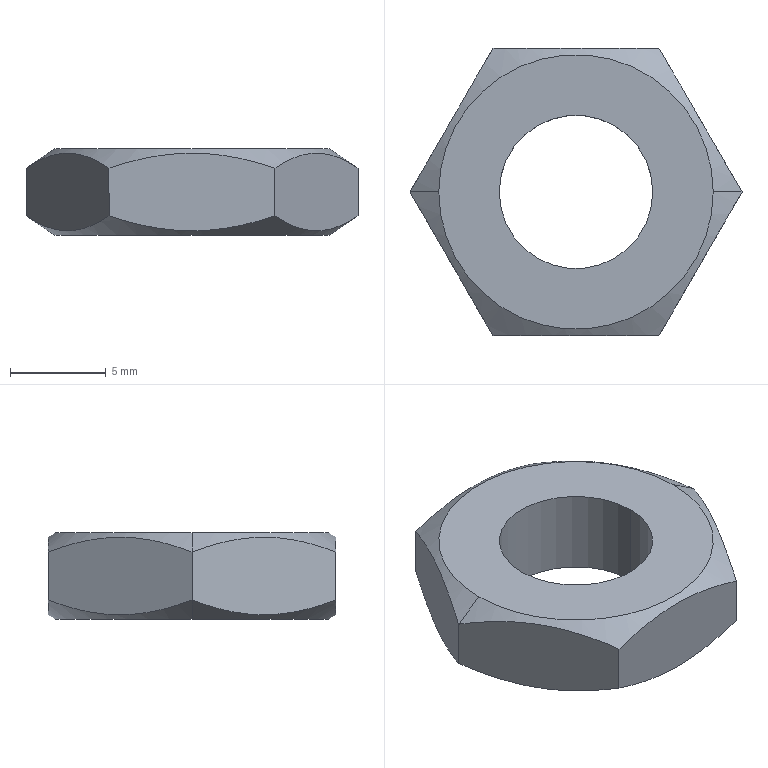Component | SolidWorks | AdjustingBoltAssembly9.26-1_M8Nut-29.26-1 | 1 solid | 14 faces | volume 630 mm3 | plane 8 | cone 4 | cylinder 2 | commonest cylinder face diameters 8 x2 | material AISI 1045 Steel, Cold Drawn